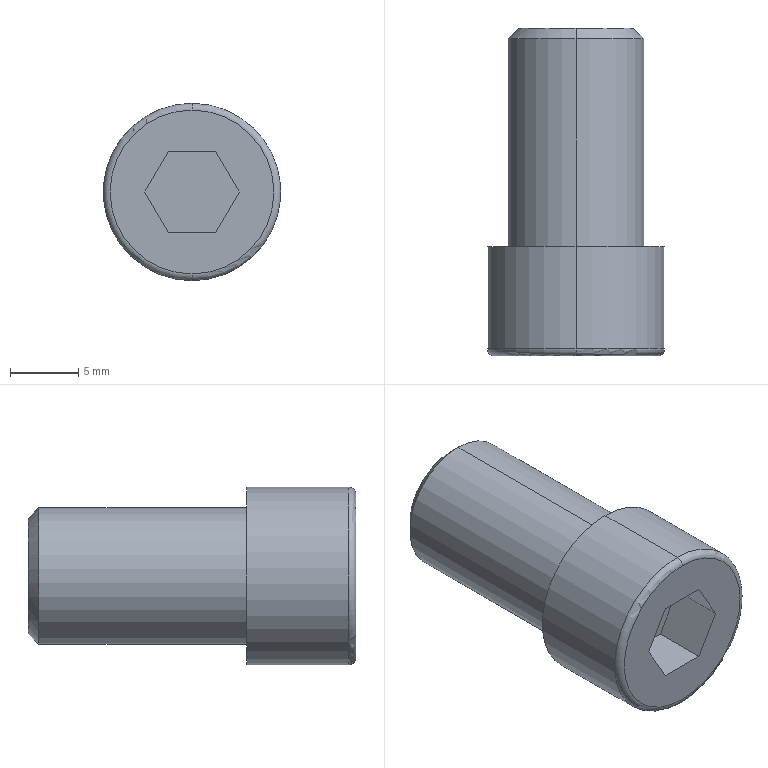Component | SolidWorks | AirTACCylinderFSC_80x75_S_FB-1_FSC_80_Screw-1 | 1 solid | 18 faces | box 13 x 24 x 13 mm | volume 2183 mm3 | plane 10 | cylinder 4 | cone 2 | torus 2 | commonest cylinder face diameters 10 x2 13 x2 | material Plain Carbon Steel
build123d program:
from build123d import *

# Parameters (mm, degrees)
CUT_EXTRUDE1_DEPTH = 4


with BuildPart() as part:
    # Sketch1 → Revolve1 (revolve)
    with BuildSketch(Plane.XY, mode=Mode.PRIVATE) as revolve1_sk:
        with BuildLine():
            Line((-8, 0), (-8, 6))
            ThreePointArc((-8, 6), (-7.854, 6.354), (-7.5, 6.5))
            Line((-7.5, 6.5), (0, 6.5))
            Line((0, 6.5), (0, 5))
            Line((0, 5), (15.233, 5))
            Line((15.233, 5), (16, 4.233))
            Line((16, 4.233), (16, 0))
            Line((16, 0), (-8, 0))
        make_face()
    revolve(revolve1_sk.sketch.rotate(Axis((16, 0, 0), (-1, 0, 0)), 270), axis=Axis((16, 0, 0), (-1, 0, 0)))

    # Sketch2 → Cut-Extrude1 (cut)
    with BuildSketch(Plane(origin=(-8, 0, 0), x_dir=(0, 0, -1), z_dir=(1, 0, 0))):
        Polygon((-3, 1.732), (-3, -1.732), (0, -3.464), (3, -1.732), (3, 1.732), (0, 3.464), align=None)
    extrude(amount=CUT_EXTRUDE1_DEPTH, mode=Mode.SUBTRACT)


solid = part.part

# Placed as in the assembly
solid = solid.moved(Location((35, 10.5, 35), (0, 0, 90)))
STEP:
#1=COLOUR_RGB('',0.7922,0.8196,0.9333);
#2=FILL_AREA_STYLE_COLOUR('',#1);
#3=FILL_AREA_STYLE('',(#2));
#4=SURFACE_STYLE_FILL_AREA(#3);
#5=SURFACE_SIDE_STYLE('',(#4));
#6=SURFACE_STYLE_USAGE(.BOTH.,#5);
#7=PRESENTATION_STYLE_ASSIGNMENT((#6));
#8=CARTESIAN_POINT('',(1.378,1.043,1.545));
#9=VERTEX_POINT('',#8);
#10=CARTESIAN_POINT('',(1.378,1.043,1.211));
#11=VERTEX_POINT('',#10);
#12=CARTESIAN_POINT('',(1.378,1.043,1.378));
#13=DIRECTION('',(0.,-1.,0.));
#14=DIRECTION('',(0.,0.,1.));
#15=AXIS2_PLACEMENT_3D('',#12,#13,#14);
#16=CIRCLE('',#15,0.1667);
#17=EDGE_CURVE('',#9,#11,#16,.T.);
#18=ORIENTED_EDGE('',*,*,#17,.T.);
#19=CARTESIAN_POINT('',(1.378,1.013,1.181));
#20=VERTEX_POINT('',#19);
#21=CARTESIAN_POINT('',(1.378,1.043,1.211));
#22=DIRECTION('',(-0.,-0.7071,-0.7071));
#23=VECTOR('',#22,39.37);
#24=LINE('',#21,#23);
#25=EDGE_CURVE('',#11,#20,#24,.T.);
#26=ORIENTED_EDGE('',*,*,#25,.T.);
#27=CARTESIAN_POINT('',(1.378,1.013,1.575));
#28=VERTEX_POINT('',#27);
#29=CARTESIAN_POINT('',(1.378,1.013,1.378));
#30=DIRECTION('',(0.,-1.,0.));
#31=DIRECTION('',(0.,0.,1.));
#32=AXIS2_PLACEMENT_3D('',#29,#30,#31);
#33=CIRCLE('',#32,0.1969);
#34=EDGE_CURVE('',#28,#20,#33,.T.);
#35=ORIENTED_EDGE('',*,*,#34,.F.);
#36=CARTESIAN_POINT('',(1.378,1.043,1.545));
#37=DIRECTION('',(0.,-0.7071,0.7071));
#38=VECTOR('',#37,39.37);
#39=LINE('',#36,#38);
#40=EDGE_CURVE('',#9,#28,#39,.T.);
#41=ORIENTED_EDGE('',*,*,#40,.F.);
#42=EDGE_LOOP('',(#18,#26,#35,#41));
#43=FACE_OUTER_BOUND('',#42,.T.);
#44=CARTESIAN_POINT('',(1.378,1.043,1.378));
#45=DIRECTION('',(0.,-1.,0.));
#46=DIRECTION('',(0.,0.,1.));
#47=AXIS2_PLACEMENT_3D('',#44,#45,#46);
#48=CONICAL_SURFACE('',#47,0.1667,0.7854);
#49=ADVANCED_FACE('',(#43),#48,.T.);
#50=ORIENTED_EDGE('',*,*,#34,.T.);
#51=CARTESIAN_POINT('',(1.378,0.4134,1.181));
#52=VERTEX_POINT('',#51);
#53=CARTESIAN_POINT('',(1.378,1.043,1.181));
#54=DIRECTION('',(0.,-1.,0.));
#55=VECTOR('',#54,39.37);
#56=LINE('',#53,#55);
#57=EDGE_CURVE('',#20,#52,#56,.T.);
#58=ORIENTED_EDGE('',*,*,#57,.T.);
#59=CARTESIAN_POINT('',(1.378,0.4134,1.575));
#60=VERTEX_POINT('',#59);
#61=CARTESIAN_POINT('',(1.378,0.4134,1.378));
#62=DIRECTION('',(0.,-1.,0.));
#63=DIRECTION('',(0.,0.,1.));
#64=AXIS2_PLACEMENT_3D('',#61,#62,#63);
#65=CIRCLE('',#64,0.1969);
#66=EDGE_CURVE('',#60,#52,#65,.T.);
#67=ORIENTED_EDGE('',*,*,#66,.F.);
#68=CARTESIAN_POINT('',(1.378,1.043,1.575));
#69=DIRECTION('',(0.,-1.,0.));
#70=VECTOR('',#69,39.37);
#71=LINE('',#68,#70);
#72=EDGE_CURVE('',#28,#60,#71,.T.);
#73=ORIENTED_EDGE('',*,*,#72,.F.);
#74=EDGE_LOOP('',(#50,#58,#67,#73));
#75=FACE_OUTER_BOUND('',#74,.T.);
#76=CARTESIAN_POINT('',(1.378,1.043,1.378));
#77=DIRECTION('',(0.,-1.,0.));
#78=DIRECTION('',(0.,0.,1.));
#79=AXIS2_PLACEMENT_3D('',#76,#77,#78);
#80=CYLINDRICAL_SURFACE('',#79,0.1969);
#81=ADVANCED_FACE('',(#75),#80,.T.);
#82=CARTESIAN_POINT('',(1.378,0.4134,1.634));
#83=VERTEX_POINT('',#82);
#84=CARTESIAN_POINT('',(1.378,0.4134,1.122));
#85=VERTEX_POINT('',#84);
#86=CARTESIAN_POINT('',(1.378,0.4134,1.378));
#87=DIRECTION('',(0.,-1.,0.));
#88=DIRECTION('',(0.,0.,1.));
#89=AXIS2_PLACEMENT_3D('',#86,#87,#88);
#90=CIRCLE('',#89,0.2559);
#91=EDGE_CURVE('',#83,#85,#90,.T.);
#92=ORIENTED_EDGE('',*,*,#91,.T.);
#93=CARTESIAN_POINT('',(1.378,0.1181,1.122));
#94=VERTEX_POINT('',#93);
#95=CARTESIAN_POINT('',(1.378,1.043,1.122));
#96=DIRECTION('',(0.,-1.,0.));
#97=VECTOR('',#96,39.37);
#98=LINE('',#95,#97);
#99=EDGE_CURVE('',#85,#94,#98,.T.);
#100=ORIENTED_EDGE('',*,*,#99,.T.);
#101=CARTESIAN_POINT('',(1.378,0.1181,1.634));
#102=VERTEX_POINT('',#101);
#103=CARTESIAN_POINT('',(1.378,0.1181,1.378));
#104=DIRECTION('',(0.,-1.,0.));
#105=DIRECTION('',(0.,0.,1.));
#106=AXIS2_PLACEMENT_3D('',#103,#104,#105);
#107=CIRCLE('',#106,0.2559);
#108=EDGE_CURVE('',#102,#94,#107,.T.);
#109=ORIENTED_EDGE('',*,*,#108,.F.);
#110=CARTESIAN_POINT('',(1.378,1.043,1.634));
#111=DIRECTION('',(0.,-1.,0.));
#112=VECTOR('',#111,39.37);
#113=LINE('',#110,#112);
#114=EDGE_CURVE('',#83,#102,#113,.T.);
#115=ORIENTED_EDGE('',*,*,#114,.F.);
#116=EDGE_LOOP('',(#92,#100,#109,#115));
#117=FACE_OUTER_BOUND('',#116,.T.);
#118=CARTESIAN_POINT('',(1.378,1.043,1.378));
#119=DIRECTION('',(0.,-1.,0.));
#120=DIRECTION('',(0.,0.,1.));
#121=AXIS2_PLACEMENT_3D('',#118,#119,#120);
#122=CYLINDRICAL_SURFACE('',#121,0.2559);
#123=ADVANCED_FACE('',(#117),#122,.T.);
#124=ORIENTED_EDGE('',*,*,#108,.T.);
#125=CARTESIAN_POINT('',(1.378,0.09843,1.142));
#126=VERTEX_POINT('',#125);
#127=CARTESIAN_POINT('',(1.378,0.1181,1.142));
#128=DIRECTION('',(-1.,0.,0.));
#129=DIRECTION('',(0.,0.,1.));
#130=AXIS2_PLACEMENT_3D('',#127,#128,#129);
#131=CIRCLE('',#130,0.01969);
#132=EDGE_CURVE('',#94,#126,#131,.T.);
#133=ORIENTED_EDGE('',*,*,#132,.T.);
#134=CARTESIAN_POINT('',(1.378,0.09843,1.614));
#135=VERTEX_POINT('',#134);
#136=CARTESIAN_POINT('',(1.378,0.09843,1.378));
#137=DIRECTION('',(0.,-1.,0.));
#138=DIRECTION('',(0.,0.,1.));
#139=AXIS2_PLACEMENT_3D('',#136,#137,#138);
#140=CIRCLE('',#139,0.2362);
#141=EDGE_CURVE('',#135,#126,#140,.T.);
#142=ORIENTED_EDGE('',*,*,#141,.F.);
#143=CARTESIAN_POINT('',(1.378,0.1181,1.614));
#144=DIRECTION('',(1.,0.,0.));
#145=DIRECTION('',(0.,0.,-1.));
#146=AXIS2_PLACEMENT_3D('',#143,#144,#145);
#147=CIRCLE('',#146,0.01969);
#148=EDGE_CURVE('',#102,#135,#147,.T.);
#149=ORIENTED_EDGE('',*,*,#148,.F.);
#150=EDGE_LOOP('',(#124,#133,#142,#149));
#151=FACE_OUTER_BOUND('',#150,.T.);
#152=CARTESIAN_POINT('',(1.378,0.1181,1.378));
#153=DIRECTION('',(0.,-1.,0.));
#154=DIRECTION('',(0.,0.,1.));
#155=AXIS2_PLACEMENT_3D('',#152,#153,#154);
#156=TOROIDAL_SURFACE('',#155,0.2362,0.01969);
#157=ADVANCED_FACE('',(#151),#156,.T.);
#158=ORIENTED_EDGE('',*,*,#141,.T.);
#159=CARTESIAN_POINT('',(1.378,0.09843,1.378));
#160=DIRECTION('',(0.,-1.,0.));
#161=DIRECTION('',(0.,0.,1.));
#162=AXIS2_PLACEMENT_3D('',#159,#160,#161);
#163=CIRCLE('',#162,0.2362);
#164=EDGE_CURVE('',#126,#135,#163,.T.);
#165=ORIENTED_EDGE('',*,*,#164,.T.);
#166=EDGE_LOOP('',(#158,#165));
#167=FACE_OUTER_BOUND('',#166,.T.);
#168=CARTESIAN_POINT('',(1.242,0.09843,1.378));
#169=VERTEX_POINT('',#168);
#170=CARTESIAN_POINT('',(1.31,0.09843,1.496));
#171=VERTEX_POINT('',#170);
#172=CARTESIAN_POINT('',(1.242,0.09843,1.378));
#173=DIRECTION('',(0.5,0.,0.866));
#174=VECTOR('',#173,39.37);
#175=LINE('',#172,#174);
#176=EDGE_CURVE('',#169,#171,#175,.T.);
#177=ORIENTED_EDGE('',*,*,#176,.T.);
#178=CARTESIAN_POINT('',(1.446,0.09843,1.496));
#179=VERTEX_POINT('',#178);
#180=CARTESIAN_POINT('',(1.31,0.09843,1.496));
#181=DIRECTION('',(1.,0.,0.));
#182=VECTOR('',#181,39.37);
#183=LINE('',#180,#182);
#184=EDGE_CURVE('',#171,#179,#183,.T.);
#185=ORIENTED_EDGE('',*,*,#184,.T.);
#186=CARTESIAN_POINT('',(1.514,0.09843,1.378));
#187=VERTEX_POINT('',#186);
#188=CARTESIAN_POINT('',(1.446,0.09843,1.496));
#189=DIRECTION('',(0.5,0.,-0.866));
#190=VECTOR('',#189,39.37);
#191=LINE('',#188,#190);
#192=EDGE_CURVE('',#179,#187,#191,.T.);
#193=ORIENTED_EDGE('',*,*,#192,.T.);
#194=CARTESIAN_POINT('',(1.446,0.09843,1.26));
#195=VERTEX_POINT('',#194);
#196=CARTESIAN_POINT('',(1.514,0.09843,1.378));
#197=DIRECTION('',(-0.5,0.,-0.866));
#198=VECTOR('',#197,39.37);
#199=LINE('',#196,#198);
#200=EDGE_CURVE('',#187,#195,#199,.T.);
#201=ORIENTED_EDGE('',*,*,#200,.T.);
#202=CARTESIAN_POINT('',(1.31,0.09843,1.26));
#203=VERTEX_POINT('',#202);
#204=CARTESIAN_POINT('',(1.446,0.09843,1.26));
#205=DIRECTION('',(-1.,0.,0.));
#206=VECTOR('',#205,39.37);
#207=LINE('',#204,#206);
#208=EDGE_CURVE('',#195,#203,#207,.T.);
#209=ORIENTED_EDGE('',*,*,#208,.T.);
#210=CARTESIAN_POINT('',(1.31,0.09843,1.26));
#211=DIRECTION('',(-0.5,0.,0.866));
#212=VECTOR('',#211,39.37);
#213=LINE('',#210,#212);
#214=EDGE_CURVE('',#203,#169,#213,.T.);
#215=ORIENTED_EDGE('',*,*,#214,.T.);
#216=EDGE_LOOP('',(#177,#185,#193,#201,#209,#215));
#217=FACE_BOUND('',#216,.T.);
#218=CARTESIAN_POINT('',(1.378,0.09843,1.378));
#219=DIRECTION('',(0.,1.,0.));
#220=DIRECTION('',(0.,0.,-1.));
#221=AXIS2_PLACEMENT_3D('',#218,#219,#220);
#222=PLANE('',#221);
#223=ADVANCED_FACE('',(#167,#217),#222,.F.);
#224=ORIENTED_EDGE('',*,*,#132,.F.);
#225=CARTESIAN_POINT('',(1.378,0.1181,1.378));
#226=DIRECTION('',(0.,-1.,0.));
#227=DIRECTION('',(0.,0.,1.));
#228=AXIS2_PLACEMENT_3D('',#225,#226,#227);
#229=CIRCLE('',#228,0.2559);
#230=EDGE_CURVE('',#94,#102,#229,.T.);
#231=ORIENTED_EDGE('',*,*,#230,.T.);
#232=ORIENTED_EDGE('',*,*,#148,.T.);
#233=ORIENTED_EDGE('',*,*,#164,.F.);
#234=EDGE_LOOP('',(#224,#231,#232,#233));
#235=FACE_OUTER_BOUND('',#234,.T.);
#236=CARTESIAN_POINT('',(1.378,0.1181,1.378));
#237=DIRECTION('',(0.,-1.,0.));
#238=DIRECTION('',(0.,0.,1.));
#239=AXIS2_PLACEMENT_3D('',#236,#237,#238);
#240=TOROIDAL_SURFACE('',#239,0.2362,0.01969);
#241=ADVANCED_FACE('',(#235),#240,.T.);
#242=ORIENTED_EDGE('',*,*,#99,.F.);
#243=CARTESIAN_POINT('',(1.378,0.4134,1.378));
#244=DIRECTION('',(0.,-1.,0.));
#245=DIRECTION('',(0.,0.,1.));
#246=AXIS2_PLACEMENT_3D('',#243,#244,#245);
#247=CIRCLE('',#246,0.2559);
#248=EDGE_CURVE('',#85,#83,#247,.T.);
#249=ORIENTED_EDGE('',*,*,#248,.T.);
#250=ORIENTED_EDGE('',*,*,#114,.T.);
#251=ORIENTED_EDGE('',*,*,#230,.F.);
#252=EDGE_LOOP('',(#242,#249,#250,#251));
#253=FACE_OUTER_BOUND('',#252,.T.);
#254=CARTESIAN_POINT('',(1.378,1.043,1.378));
#255=DIRECTION('',(0.,-1.,0.));
#256=DIRECTION('',(0.,0.,1.));
#257=AXIS2_PLACEMENT_3D('',#254,#255,#256);
#258=CYLINDRICAL_SURFACE('',#257,0.2559);
#259=ADVANCED_FACE('',(#253),#258,.T.);
#260=ORIENTED_EDGE('',*,*,#91,.F.);
#261=ORIENTED_EDGE('',*,*,#248,.F.);
#262=EDGE_LOOP('',(#260,#261));
#263=FACE_OUTER_BOUND('',#262,.T.);
#264=ORIENTED_EDGE('',*,*,#66,.T.);
#265=CARTESIAN_POINT('',(1.378,0.4134,1.378));
#266=DIRECTION('',(0.,-1.,0.));
#267=DIRECTION('',(0.,0.,1.));
#268=AXIS2_PLACEMENT_3D('',#265,#266,#267);
#269=CIRCLE('',#268,0.1969);
#270=EDGE_CURVE('',#52,#60,#269,.T.);
#271=ORIENTED_EDGE('',*,*,#270,.T.);
#272=EDGE_LOOP('',(#264,#271));
#273=FACE_BOUND('',#272,.T.);
#274=CARTESIAN_POINT('',(1.122,0.4134,1.378));
#275=DIRECTION('',(0.,-1.,0.));
#276=DIRECTION('',(0.,0.,1.));
#277=AXIS2_PLACEMENT_3D('',#274,#275,#276);
#278=PLANE('',#277);
#279=ADVANCED_FACE('',(#263,#273),#278,.F.);
#280=ORIENTED_EDGE('',*,*,#57,.F.);
#281=CARTESIAN_POINT('',(1.378,1.013,1.378));
#282=DIRECTION('',(0.,-1.,0.));
#283=DIRECTION('',(0.,0.,1.));
#284=AXIS2_PLACEMENT_3D('',#281,#282,#283);
#285=CIRCLE('',#284,0.1969);
#286=EDGE_CURVE('',#20,#28,#285,.T.);
#287=ORIENTED_EDGE('',*,*,#286,.T.);
#288=ORIENTED_EDGE('',*,*,#72,.T.);
#289=ORIENTED_EDGE('',*,*,#270,.F.);
#290=EDGE_LOOP('',(#280,#287,#288,#289));
#291=FACE_OUTER_BOUND('',#290,.T.);
#292=CARTESIAN_POINT('',(1.378,1.043,1.378));
#293=DIRECTION('',(0.,-1.,0.));
#294=DIRECTION('',(0.,0.,1.));
#295=AXIS2_PLACEMENT_3D('',#292,#293,#294);
#296=CYLINDRICAL_SURFACE('',#295,0.1969);
#297=ADVANCED_FACE('',(#291),#296,.T.);
#298=ORIENTED_EDGE('',*,*,#25,.F.);
#299=CARTESIAN_POINT('',(1.378,1.043,1.378));
#300=DIRECTION('',(0.,-1.,0.));
#301=DIRECTION('',(0.,0.,1.));
#302=AXIS2_PLACEMENT_3D('',#299,#300,#301);
#303=CIRCLE('',#302,0.1667);
#304=EDGE_CURVE('',#11,#9,#303,.T.);
#305=ORIENTED_EDGE('',*,*,#304,.T.);
#306=ORIENTED_EDGE('',*,*,#40,.T.);
#307=ORIENTED_EDGE('',*,*,#286,.F.);
#308=EDGE_LOOP('',(#298,#305,#306,#307));
#309=FACE_OUTER_BOUND('',#308,.T.);
#310=CARTESIAN_POINT('',(1.378,1.043,1.378));
#311=DIRECTION('',(0.,-1.,0.));
#312=DIRECTION('',(0.,0.,1.));
#313=AXIS2_PLACEMENT_3D('',#310,#311,#312);
#314=CONICAL_SURFACE('',#313,0.1667,0.7854);
#315=ADVANCED_FACE('',(#309),#314,.T.);
#316=ORIENTED_EDGE('',*,*,#17,.F.);
#317=ORIENTED_EDGE('',*,*,#304,.F.);
#318=EDGE_LOOP('',(#316,#317));
#319=FACE_OUTER_BOUND('',#318,.T.);
#320=CARTESIAN_POINT('',(1.211,1.043,1.378));
#321=DIRECTION('',(0.,-1.,0.));
#322=DIRECTION('',(0.,0.,1.));
#323=AXIS2_PLACEMENT_3D('',#320,#321,#322);
#324=PLANE('',#323);
#325=ADVANCED_FACE('',(#319),#324,.F.);
#326=ORIENTED_EDGE('',*,*,#176,.F.);
#327=CARTESIAN_POINT('',(1.242,0.2559,1.378));
#328=VERTEX_POINT('',#327);
#329=CARTESIAN_POINT('',(1.242,0.2559,1.378));
#330=DIRECTION('',(0.,-1.,0.));
#331=VECTOR('',#330,39.37);
#332=LINE('',#329,#331);
#333=EDGE_CURVE('',#328,#169,#332,.T.);
#334=ORIENTED_EDGE('',*,*,#333,.F.);
#335=CARTESIAN_POINT('',(1.31,0.2559,1.496));
#336=VERTEX_POINT('',#335);
#337=CARTESIAN_POINT('',(1.242,0.2559,1.378));
#338=DIRECTION('',(0.5,0.,0.866));
#339=VECTOR('',#338,39.37);
#340=LINE('',#337,#339);
#341=EDGE_CURVE('',#328,#336,#340,.T.);
#342=ORIENTED_EDGE('',*,*,#341,.T.);
#343=CARTESIAN_POINT('',(1.31,0.2559,1.496));
#344=DIRECTION('',(0.,-1.,0.));
#345=VECTOR('',#344,39.37);
#346=LINE('',#343,#345);
#347=EDGE_CURVE('',#336,#171,#346,.T.);
#348=ORIENTED_EDGE('',*,*,#347,.T.);
#349=EDGE_LOOP('',(#326,#334,#342,#348));
#350=FACE_OUTER_BOUND('',#349,.T.);
#351=CARTESIAN_POINT('',(1.242,0.2559,1.378));
#352=DIRECTION('',(0.866,0.,-0.5));
#353=DIRECTION('',(-0.5,0.,-0.866));
#354=AXIS2_PLACEMENT_3D('',#351,#352,#353);
#355=PLANE('',#354);
#356=ADVANCED_FACE('',(#350),#355,.T.);
#357=ORIENTED_EDGE('',*,*,#184,.F.);
#358=ORIENTED_EDGE('',*,*,#347,.F.);
#359=CARTESIAN_POINT('',(1.446,0.2559,1.496));
#360=VERTEX_POINT('',#359);
#361=CARTESIAN_POINT('',(1.31,0.2559,1.496));
#362=DIRECTION('',(1.,0.,0.));
#363=VECTOR('',#362,39.37);
#364=LINE('',#361,#363);
#365=EDGE_CURVE('',#336,#360,#364,.T.);
#366=ORIENTED_EDGE('',*,*,#365,.T.);
#367=CARTESIAN_POINT('',(1.446,0.2559,1.496));
#368=DIRECTION('',(0.,-1.,0.));
#369=VECTOR('',#368,39.37);
#370=LINE('',#367,#369);
#371=EDGE_CURVE('',#360,#179,#370,.T.);
#372=ORIENTED_EDGE('',*,*,#371,.T.);
#373=EDGE_LOOP('',(#357,#358,#366,#372));
#374=FACE_OUTER_BOUND('',#373,.T.);
#375=CARTESIAN_POINT('',(1.31,0.2559,1.496));
#376=DIRECTION('',(0.,0.,-1.));
#377=DIRECTION('',(0.,-1.,0.));
#378=AXIS2_PLACEMENT_3D('',#375,#376,#377);
#379=PLANE('',#378);
#380=ADVANCED_FACE('',(#374),#379,.T.);
#381=ORIENTED_EDGE('',*,*,#192,.F.);
#382=ORIENTED_EDGE('',*,*,#371,.F.);
#383=CARTESIAN_POINT('',(1.514,0.2559,1.378));
#384=VERTEX_POINT('',#383);
#385=CARTESIAN_POINT('',(1.446,0.2559,1.496));
#386=DIRECTION('',(0.5,0.,-0.866));
#387=VECTOR('',#386,39.37);
#388=LINE('',#385,#387);
#389=EDGE_CURVE('',#360,#384,#388,.T.);
#390=ORIENTED_EDGE('',*,*,#389,.T.);
#391=CARTESIAN_POINT('',(1.514,0.2559,1.378));
#392=DIRECTION('',(0.,-1.,0.));
#393=VECTOR('',#392,39.37);
#394=LINE('',#391,#393);
#395=EDGE_CURVE('',#384,#187,#394,.T.);
#396=ORIENTED_EDGE('',*,*,#395,.T.);
#397=EDGE_LOOP('',(#381,#382,#390,#396));
#398=FACE_OUTER_BOUND('',#397,.T.);
#399=CARTESIAN_POINT('',(1.446,0.2559,1.496));
#400=DIRECTION('',(-0.866,0.,-0.5));
#401=DIRECTION('',(-0.5,0.,0.866));
#402=AXIS2_PLACEMENT_3D('',#399,#400,#401);
#403=PLANE('',#402);
#404=ADVANCED_FACE('',(#398),#403,.T.);
#405=ORIENTED_EDGE('',*,*,#200,.F.);
#406=ORIENTED_EDGE('',*,*,#395,.F.);
#407=CARTESIAN_POINT('',(1.446,0.2559,1.26));
#408=VERTEX_POINT('',#407);
#409=CARTESIAN_POINT('',(1.514,0.2559,1.378));
#410=DIRECTION('',(-0.5,0.,-0.866));
#411=VECTOR('',#410,39.37);
#412=LINE('',#409,#411);
#413=EDGE_CURVE('',#384,#408,#412,.T.);
#414=ORIENTED_EDGE('',*,*,#413,.T.);
#415=CARTESIAN_POINT('',(1.446,0.2559,1.26));
#416=DIRECTION('',(0.,-1.,0.));
#417=VECTOR('',#416,39.37);
#418=LINE('',#415,#417);
#419=EDGE_CURVE('',#408,#195,#418,.T.);
#420=ORIENTED_EDGE('',*,*,#419,.T.);
#421=EDGE_LOOP('',(#405,#406,#414,#420));
#422=FACE_OUTER_BOUND('',#421,.T.);
#423=CARTESIAN_POINT('',(1.514,0.2559,1.378));
#424=DIRECTION('',(-0.866,0.,0.5));
#425=DIRECTION('',(0.5,0.,0.866));
#426=AXIS2_PLACEMENT_3D('',#423,#424,#425);
#427=PLANE('',#426);
#428=ADVANCED_FACE('',(#422),#427,.T.);
#429=ORIENTED_EDGE('',*,*,#208,.F.);
#430=ORIENTED_EDGE('',*,*,#419,.F.);
#431=CARTESIAN_POINT('',(1.31,0.2559,1.26));
#432=VERTEX_POINT('',#431);
#433=CARTESIAN_POINT('',(1.446,0.2559,1.26));
#434=DIRECTION('',(-1.,0.,0.));
#435=VECTOR('',#434,39.37);
#436=LINE('',#433,#435);
#437=EDGE_CURVE('',#408,#432,#436,.T.);
#438=ORIENTED_EDGE('',*,*,#437,.T.);
#439=CARTESIAN_POINT('',(1.31,0.2559,1.26));
#440=DIRECTION('',(0.,-1.,0.));
#441=VECTOR('',#440,39.37);
#442=LINE('',#439,#441);
#443=EDGE_CURVE('',#432,#203,#442,.T.);
#444=ORIENTED_EDGE('',*,*,#443,.T.);
#445=EDGE_LOOP('',(#429,#430,#438,#444));
#446=FACE_OUTER_BOUND('',#445,.T.);
#447=CARTESIAN_POINT('',(1.446,0.2559,1.26));
#448=DIRECTION('',(0.,0.,1.));
#449=DIRECTION('',(0.,1.,0.));
#450=AXIS2_PLACEMENT_3D('',#447,#448,#449);
#451=PLANE('',#450);
#452=ADVANCED_FACE('',(#446),#451,.T.);
#453=ORIENTED_EDGE('',*,*,#214,.F.);
#454=ORIENTED_EDGE('',*,*,#443,.F.);
#455=CARTESIAN_POINT('',(1.31,0.2559,1.26));
#456=DIRECTION('',(-0.5,0.,0.866));
#457=VECTOR('',#456,39.37);
#458=LINE('',#455,#457);
#459=EDGE_CURVE('',#432,#328,#458,.T.);
#460=ORIENTED_EDGE('',*,*,#459,.T.);
#461=ORIENTED_EDGE('',*,*,#333,.T.);
#462=EDGE_LOOP('',(#453,#454,#460,#461));
#463=FACE_OUTER_BOUND('',#462,.T.);
#464=CARTESIAN_POINT('',(1.31,0.2559,1.26));
#465=DIRECTION('',(0.866,0.,0.5));
#466=DIRECTION('',(0.5,0.,-0.866));
#467=AXIS2_PLACEMENT_3D('',#464,#465,#466);
#468=PLANE('',#467);
#469=ADVANCED_FACE('',(#463),#468,.T.);
#470=ORIENTED_EDGE('',*,*,#341,.F.);
#471=ORIENTED_EDGE('',*,*,#459,.F.);
#472=ORIENTED_EDGE('',*,*,#437,.F.);
#473=ORIENTED_EDGE('',*,*,#413,.F.);
#474=ORIENTED_EDGE('',*,*,#389,.F.);
#475=ORIENTED_EDGE('',*,*,#365,.F.);
#476=EDGE_LOOP('',(#470,#471,#472,#473,#474,#475));
#477=FACE_OUTER_BOUND('',#476,.T.);
#478=CARTESIAN_POINT('',(1.31,0.2559,1.496));
#479=DIRECTION('',(0.,1.,0.));
#480=DIRECTION('',(0.,0.,-1.));
#481=AXIS2_PLACEMENT_3D('',#478,#479,#480);
#482=PLANE('',#481);
#483=ADVANCED_FACE('',(#477),#482,.F.);
#484=CLOSED_SHELL('',(#49,#81,#123,#157,#223,#241,#259,#279,#297,#315,#325,#356,#380,#404,#428,#452,#469,#483));
#485=MANIFOLD_SOLID_BREP('',#484);
#486=STYLED_ITEM('',(#7),#485);
#487=(LENGTH_UNIT()NAMED_UNIT(*)SI_UNIT($,.METRE.));
#488=LENGTH_MEASURE_WITH_UNIT(LENGTH_MEASURE(0.0254),#487);
#489=DIMENSIONAL_EXPONENTS(1.,0.,0.,0.,0.,0.,0.);
#490=(CONVERSION_BASED_UNIT('',#488)LENGTH_UNIT()NAMED_UNIT(#489));
#491=UNCERTAINTY_MEASURE_WITH_UNIT(LENGTH_MEASURE(0.00001),#490,'','');
#492=(NAMED_UNIT(*)PLANE_ANGLE_UNIT()SI_UNIT($,.RADIAN.));
#493=(NAMED_UNIT(*)SI_UNIT($,.STERADIAN.)SOLID_ANGLE_UNIT());
#494=(GEOMETRIC_REPRESENTATION_CONTEXT(3)GLOBAL_UNCERTAINTY_ASSIGNED_CONTEXT((#491))GLOBAL_UNIT_ASSIGNED_CONTEXT((#490,#492,#493))REPRESENTATION_CONTEXT('',''));
#495=MECHANICAL_DESIGN_GEOMETRIC_PRESENTATION_REPRESENTATION('',(#486),#494);
#496=CARTESIAN_POINT('',(0.,0.,0.));
#497=DIRECTION('',(0.,0.,1.));
#498=DIRECTION('',(1.,0.,0.));
#499=AXIS2_PLACEMENT_3D('',#496,#497,#498);
#500=(LENGTH_UNIT()NAMED_UNIT(*)SI_UNIT($,.METRE.));
#501=LENGTH_MEASURE_WITH_UNIT(LENGTH_MEASURE(0.0254),#500);
#502=DIMENSIONAL_EXPONENTS(1.,0.,0.,0.,0.,0.,0.);
#503=(CONVERSION_BASED_UNIT('',#501)LENGTH_UNIT()NAMED_UNIT(#502));
#504=UNCERTAINTY_MEASURE_WITH_UNIT(LENGTH_MEASURE(0.00001),#503,'','');
#505=(NAMED_UNIT(*)PLANE_ANGLE_UNIT()SI_UNIT($,.RADIAN.));
#506=(NAMED_UNIT(*)SI_UNIT($,.STERADIAN.)SOLID_ANGLE_UNIT());
#507=(GEOMETRIC_REPRESENTATION_CONTEXT(3)GLOBAL_UNCERTAINTY_ASSIGNED_CONTEXT((#504))GLOBAL_UNIT_ASSIGNED_CONTEXT((#503,#505,#506))REPRESENTATION_CONTEXT('',''));
#508=ADVANCED_BREP_SHAPE_REPRESENTATION('',(#485,#499),#507);
#509=PRESENTATION_LAYER_ASSIGNMENT('','',(#486));